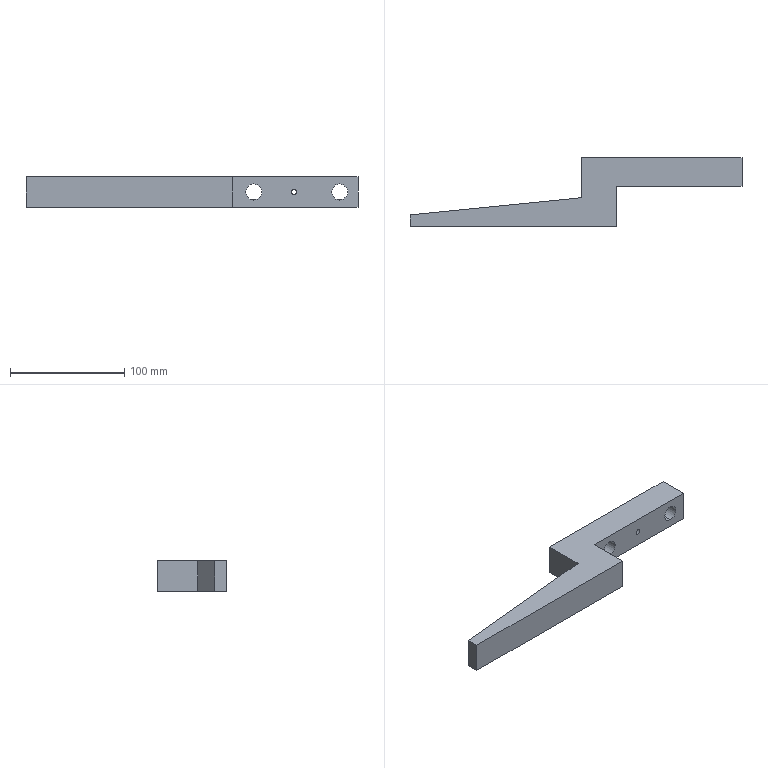Component | SolidWorks | SHYTJ-01-07-05BlankingBlock1-2-1 | 1 solid | 31 faces | box 290 x 60 x 27 mm | volume 183398 mm3 | cylinder 16 | plane 13 | cone 2 | commonest cylinder face diameters 4.2 x4 18 x4 14 x4 10 x2 8.8 x2
build123d program:
from build123d import *

# Parameters (mm, degrees)
BOSS_EXTRUDE1_DEPTH         = 27
SKETCH5_W                   = 125.175
SKETCH5_H                   = 38.879
CUT_EXTRUDE1_DEPTH          = 30
SKETCH6_R                   = 7
CUT_EXTRUDE2_2_DEPTH        = 298.37
SKETCH7_R                   = 9
CUT_EXTRUDE3_DEPTH          = 3
M5_TAPPED_HOLE1_D           = 4.2
M5_TAPPED_HOLE1_DEPTH       = 12.4
M5_TAPPED_HOLE1_TIP         = 1.262
M10X1_25_TAPPED_HOLE1_D     = 8.8
M10X1_25_TAPPED_HOLE1_DEPTH = 23.75
M10X1_25_TAPPED_HOLE1_TIP   = 2.644
CUT_EXTRUDE2_START          = 40
SKETCH2_R                   = 5
CUT_EXTRUDE2_DEPTH          = 20.5


with BuildPart() as part:
    # Sketch1 → Boss-Extrude1 (new body)
    with BuildSketch(Plane.XY):
        Polygon((0, 0), (0, 60), (140, 60), (140, 25), (290, 10), (290, 0), align=None)
    extrude(amount=BOSS_EXTRUDE1_DEPTH)

    # Sketch5 → Cut-Extrude1 (cut)
    with BuildSketch(Plane(origin=(0, 0, 0), x_dir=(-1, 0, 0), z_dir=(0, 0, -1))):
        with Locations((-47.412, 15.561)):
            Rectangle(SKETCH5_W, SKETCH5_H)
    extrude(amount=-CUT_EXTRUDE1_DEPTH, mode=Mode.SUBTRACT)

    # Sketch6 → Cut-Extrude2_2 (cut, through all)
    with BuildSketch(Plane(origin=(0, 60, 0), x_dir=(1, 0, 0), z_dir=(0, 1, 0))):
        with Locations(Location((16, -13.5, 0), (0, 0, 270))):
            Circle(SKETCH6_R)
        with Locations(Location((91, -13.5, 0), (0, 0, 270))):
            Circle(SKETCH6_R)
    extrude(amount=-CUT_EXTRUDE2_2_DEPTH, mode=Mode.SUBTRACT)

    # Sketch7 → Cut-Extrude3 (cut)
    with BuildSketch(Plane(origin=(0, 60, 0), x_dir=(1, 0, 0), z_dir=(0, 1, 0))):
        with Locations(Location((91, -13.5, 0), (0, 0, 270))):
            Circle(SKETCH7_R)
        with Locations(Location((16, -13.5, 0), (0, 0, 270))):
            Circle(SKETCH7_R)
    extrude(amount=-CUT_EXTRUDE3_DEPTH, mode=Mode.SUBTRACT)

    # M5 Tapped Hole1
    with Locations(Plane.XY.offset(27)):
        with Locations((16, 47.5), (91, 47.5)):
            Hole(M5_TAPPED_HOLE1_D / 2, depth=M5_TAPPED_HOLE1_DEPTH)
            with Locations((0, 0, -(M5_TAPPED_HOLE1_DEPTH + M5_TAPPED_HOLE1_TIP / 2))):  # 118° drill point
                Cone(0, M5_TAPPED_HOLE1_D / 2, M5_TAPPED_HOLE1_TIP, mode=Mode.SUBTRACT)

    # M10x1.25 Tapped Hole1
    with Locations(Plane(origin=(0, 60, 0), x_dir=(1, 0, 0), z_dir=(0, 1, 0))):
        with Locations((56, -13.5)):
            Hole(M10X1_25_TAPPED_HOLE1_D / 2, depth=M10X1_25_TAPPED_HOLE1_DEPTH)
            with Locations((0, 0, -(M10X1_25_TAPPED_HOLE1_DEPTH + M10X1_25_TAPPED_HOLE1_TIP / 2))):  # 118° drill point
                Cone(0, M10X1_25_TAPPED_HOLE1_D / 2, M10X1_25_TAPPED_HOLE1_TIP, mode=Mode.SUBTRACT)

    # Sketch2 → Cut-Extrude2 (cut)
    with BuildSketch(Plane(origin=(0, 0, 0), x_dir=(1, 0, 0), z_dir=(0, 1, 0)).offset(CUT_EXTRUDE2_START)):
        with Locations(Location((56, -13.5, 0), (0, 0, 90))):
            Circle(SKETCH2_R)
    extrude(amount=CUT_EXTRUDE2_DEPTH, mode=Mode.SUBTRACT)


solid = part.part

# Placed as in the assembly
solid = solid.moved(Location((230.884, -144.361, 283.5), (-180, 0, 180)))